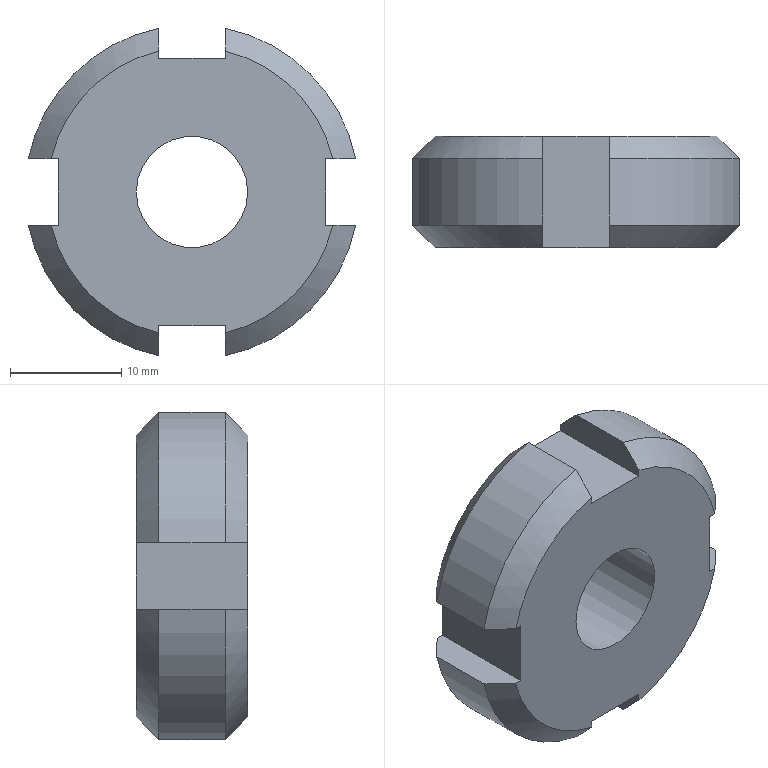Component | NX | NUT_M10 | 1 solid | 27 faces | volume 5322 mm3 | plane 14 | cone 8 | cylinder 5 | commonest cylinder face diameters 30 x4 10 x1